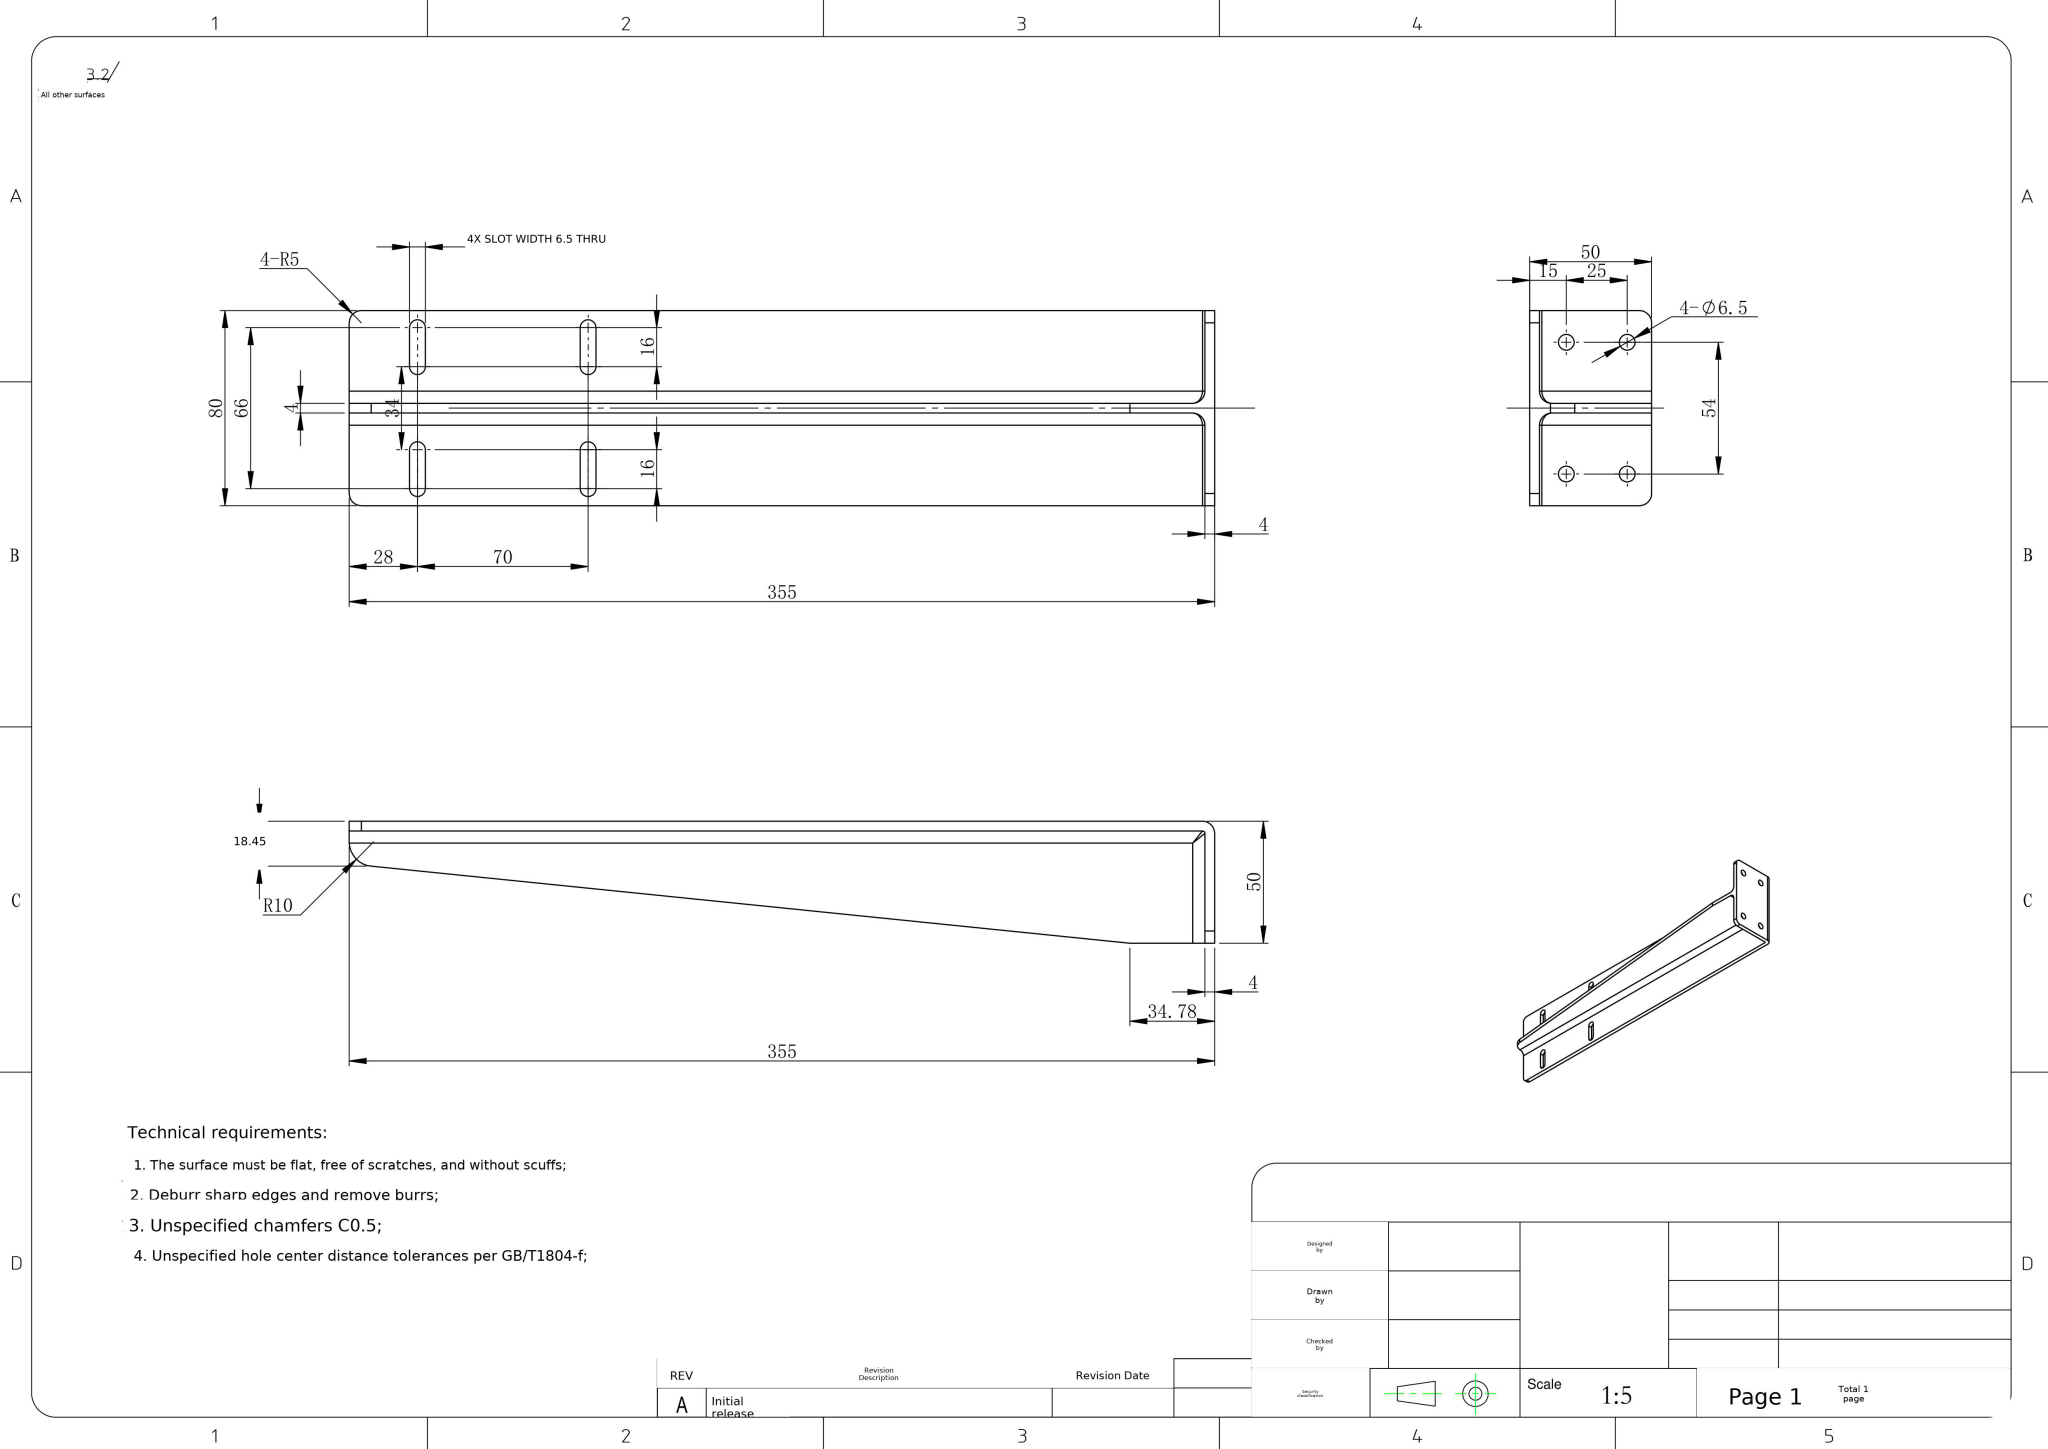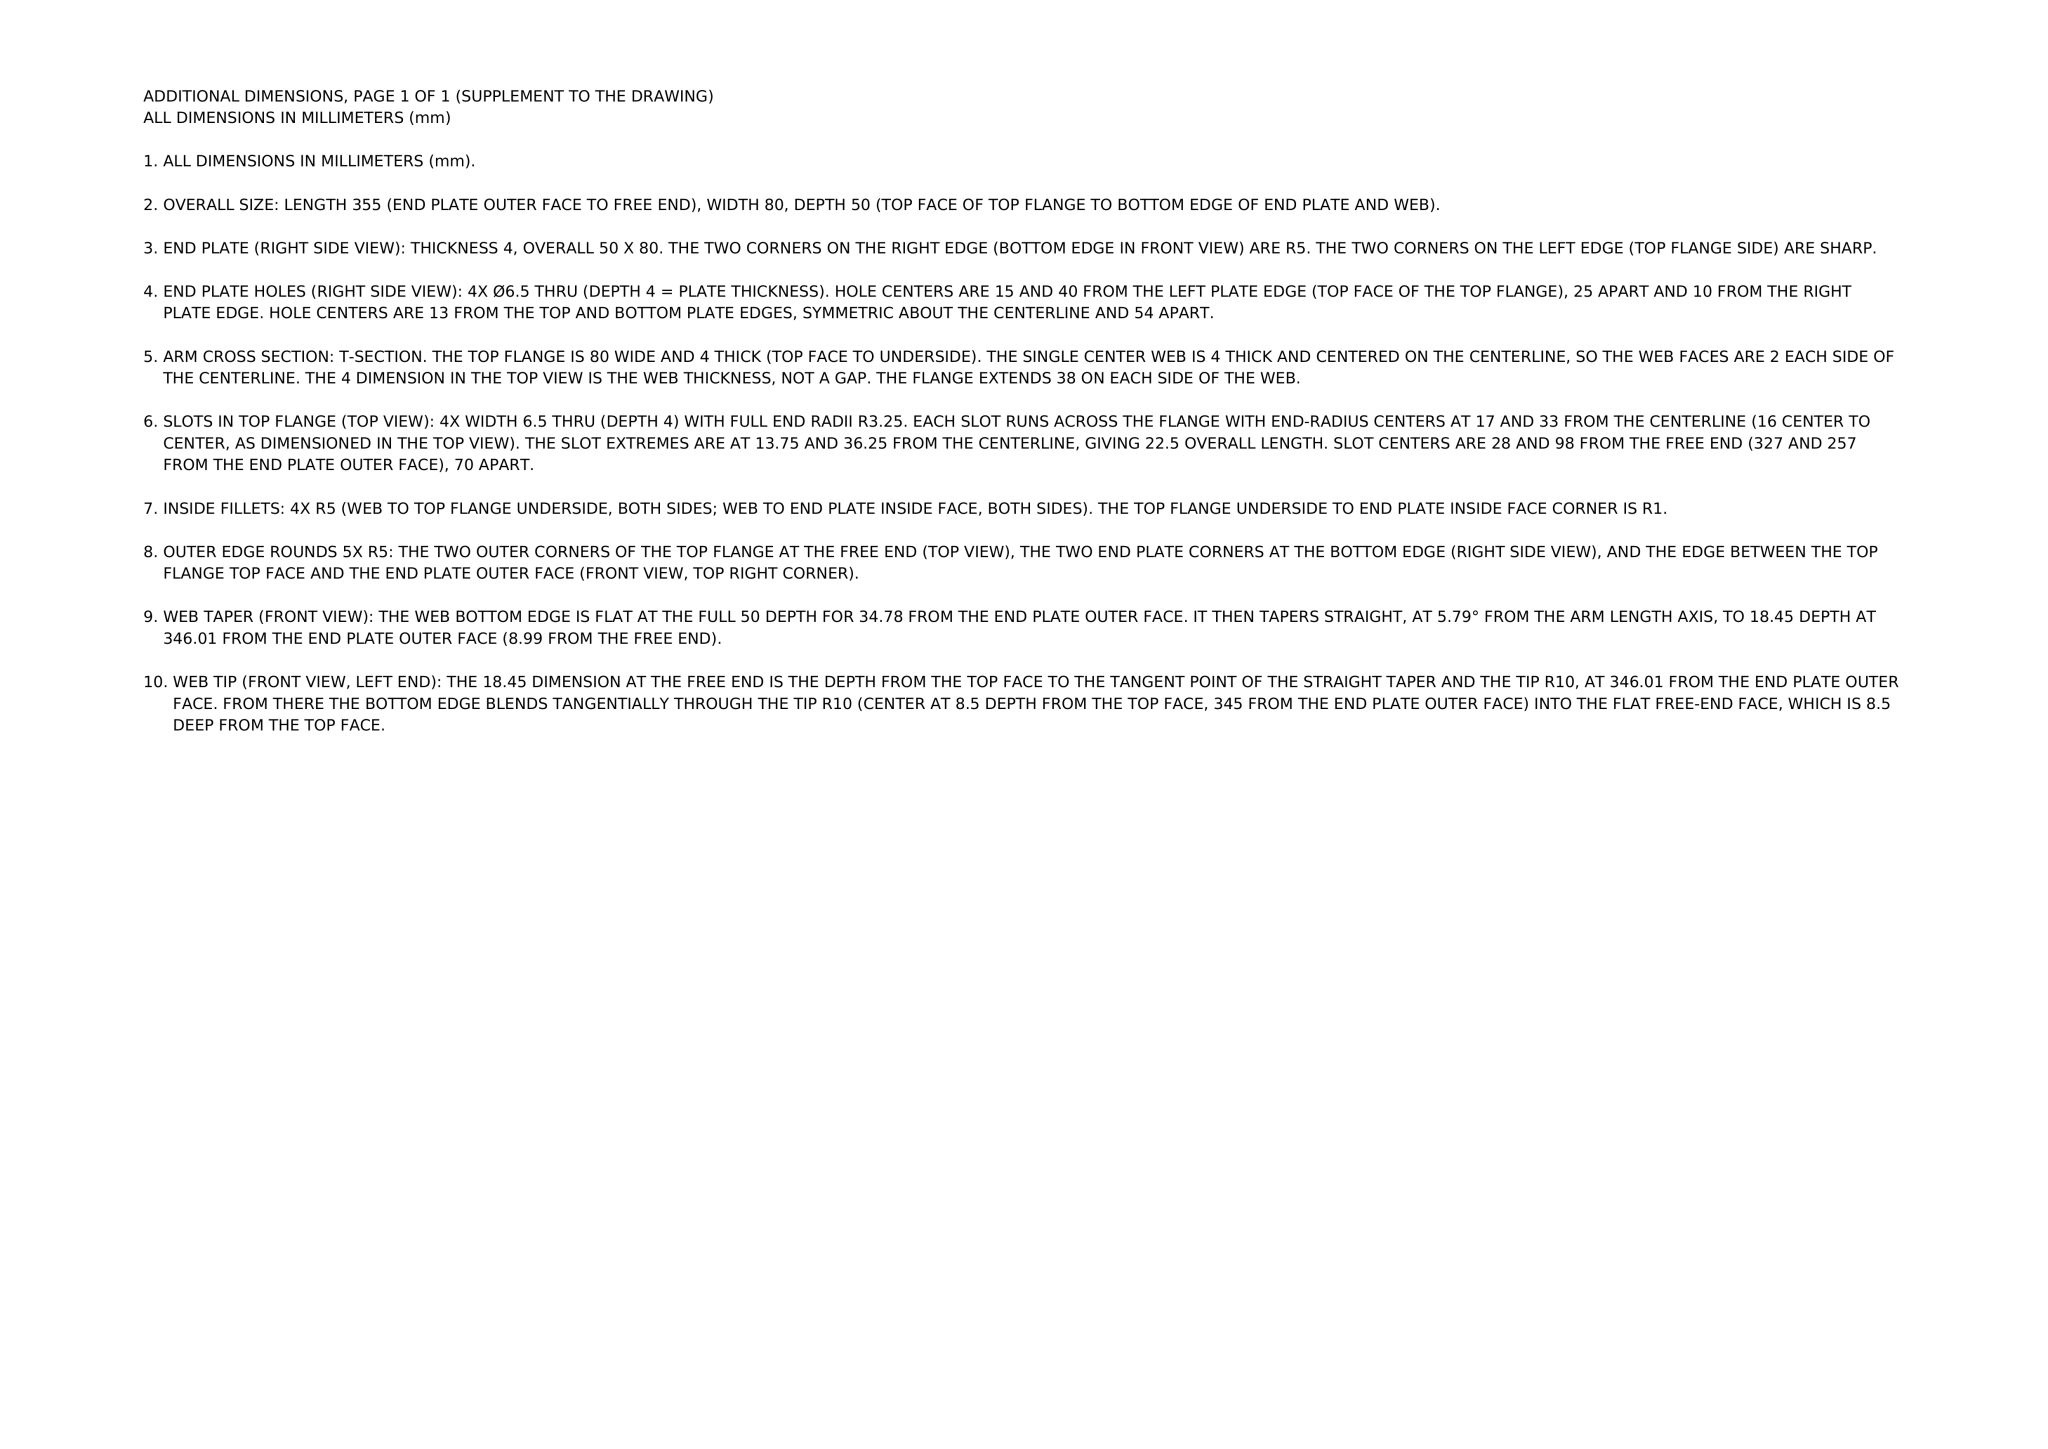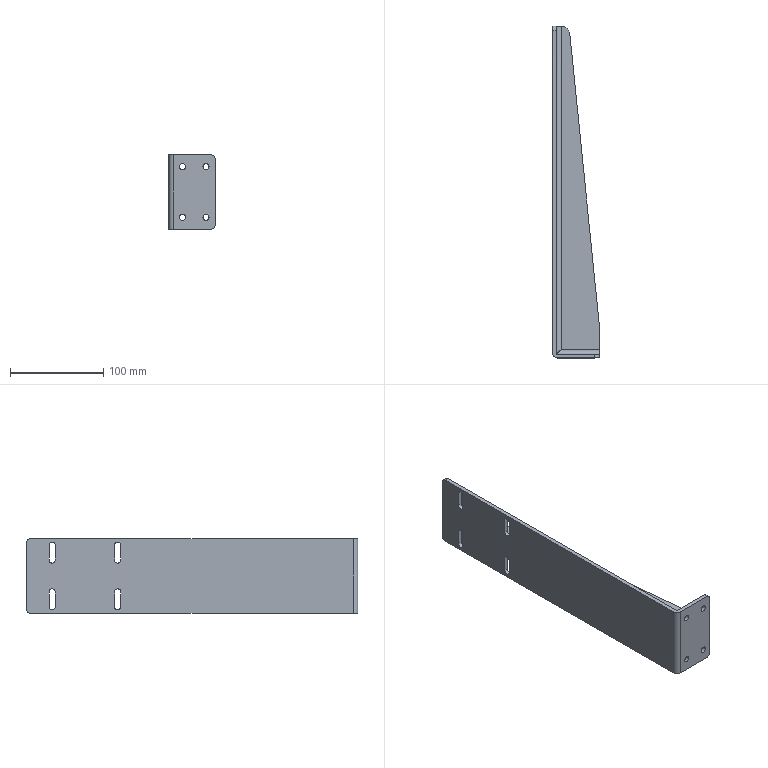Part | NX | mm | 1 solid | 55 faces | box 50 x 355 x 80 mm | volume 173055 mm3 | cylinder 32 | plane 21 | spline 2 | commonest cylinder face diameters 6.5 x20 10 x9 2 x2 20 x1